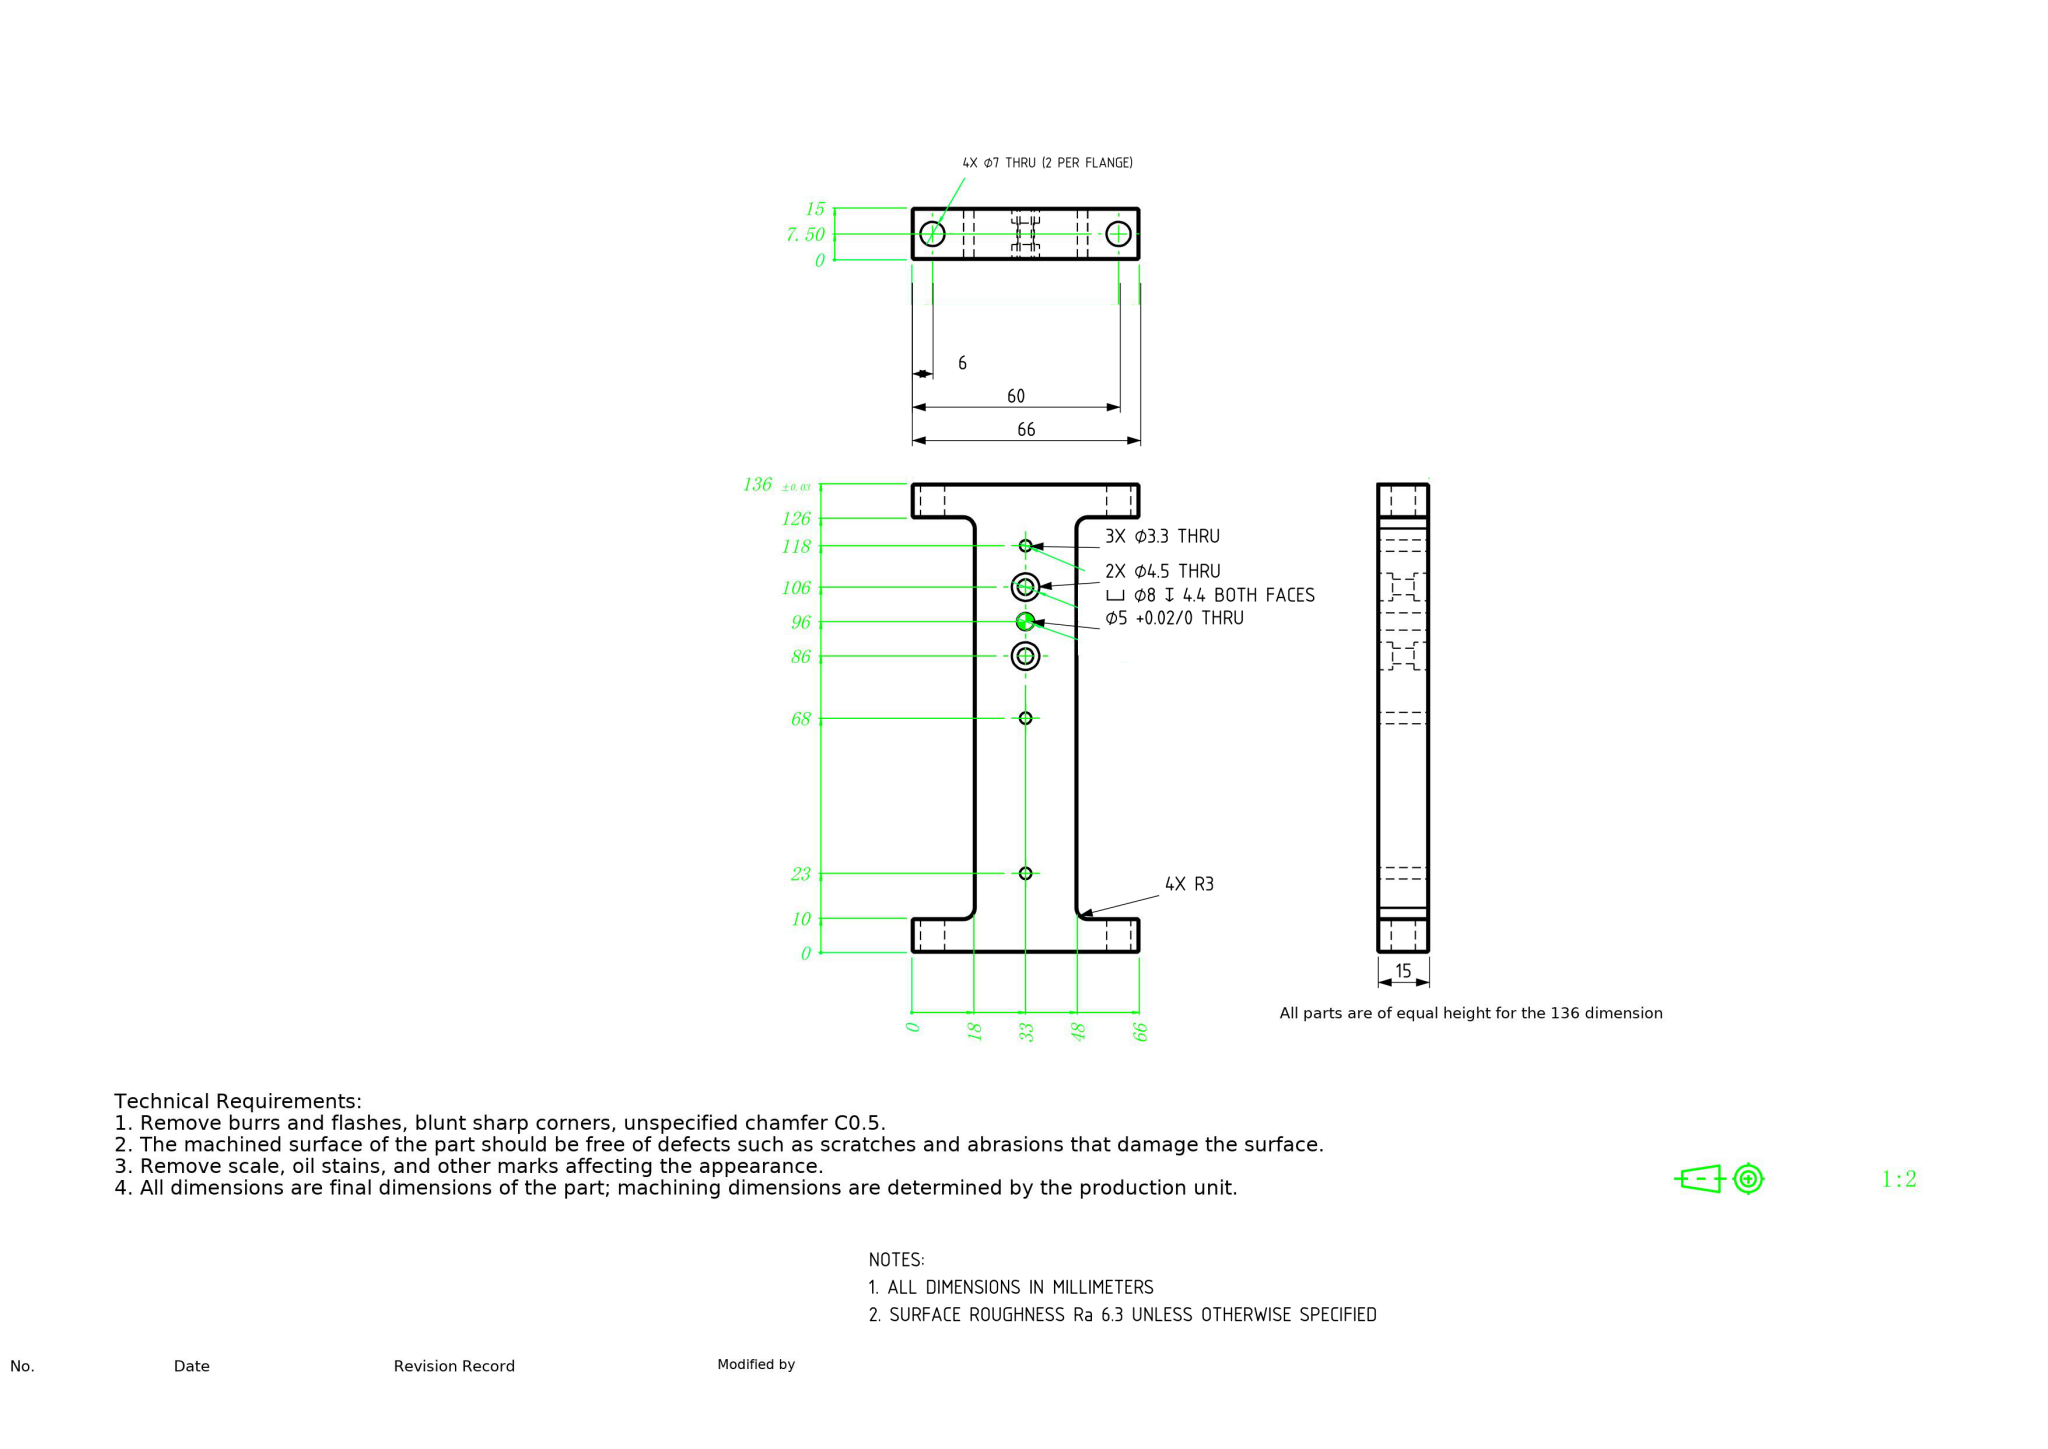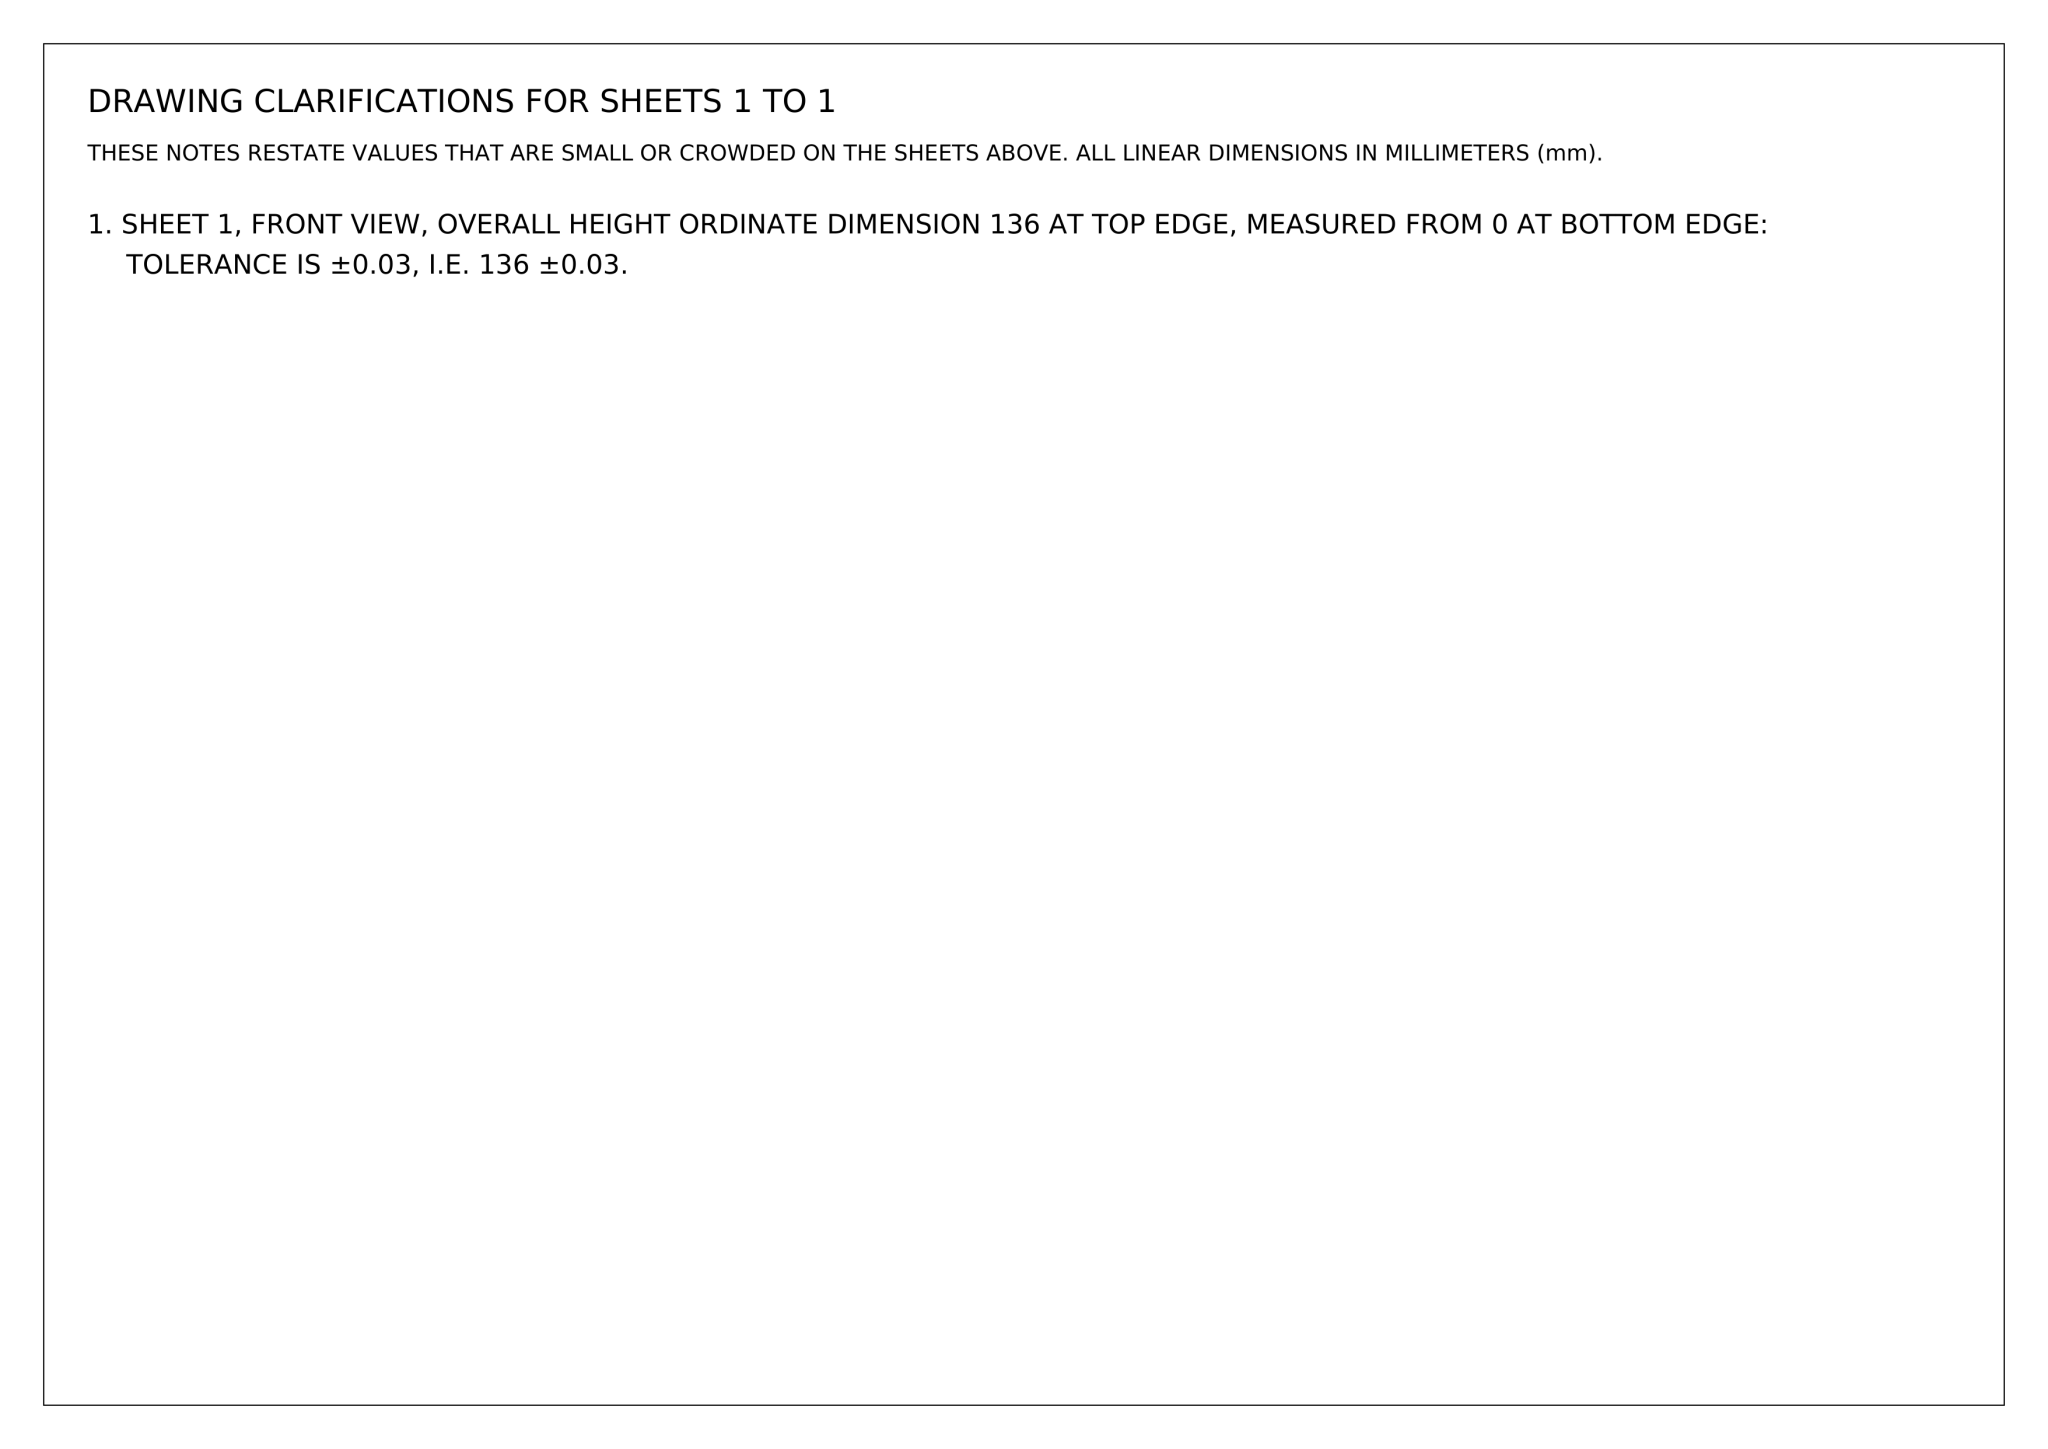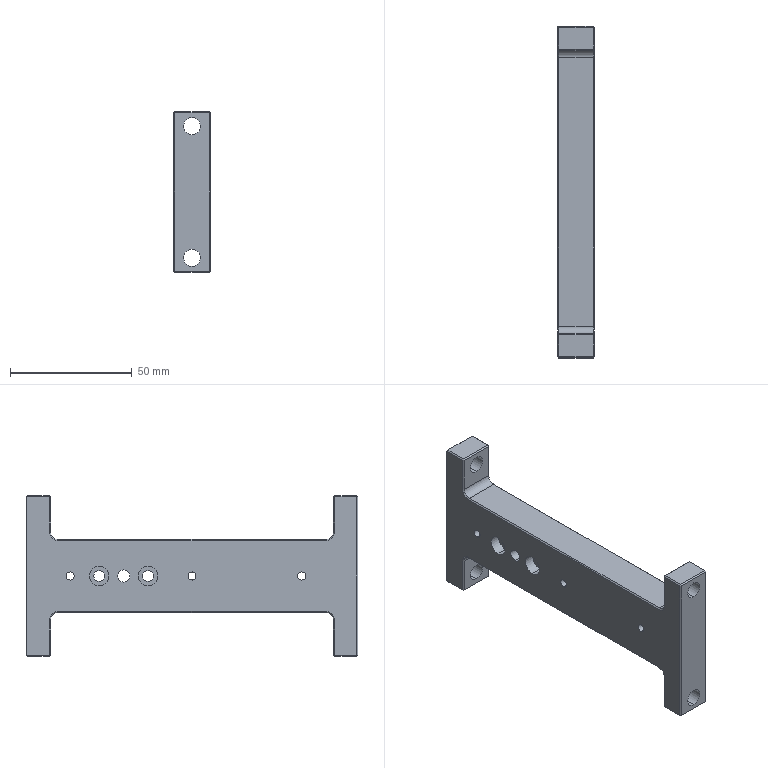Part | NX | mm | 1 solid | 103 faces | box 15 x 136 x 66 mm | volume 68692 mm3 | plane 63 | cylinder 32 | cone 8 | commonest cylinder face diameters 8 x8 7 x8 3.3 x6 4.5 x4 6 x4 5 x2